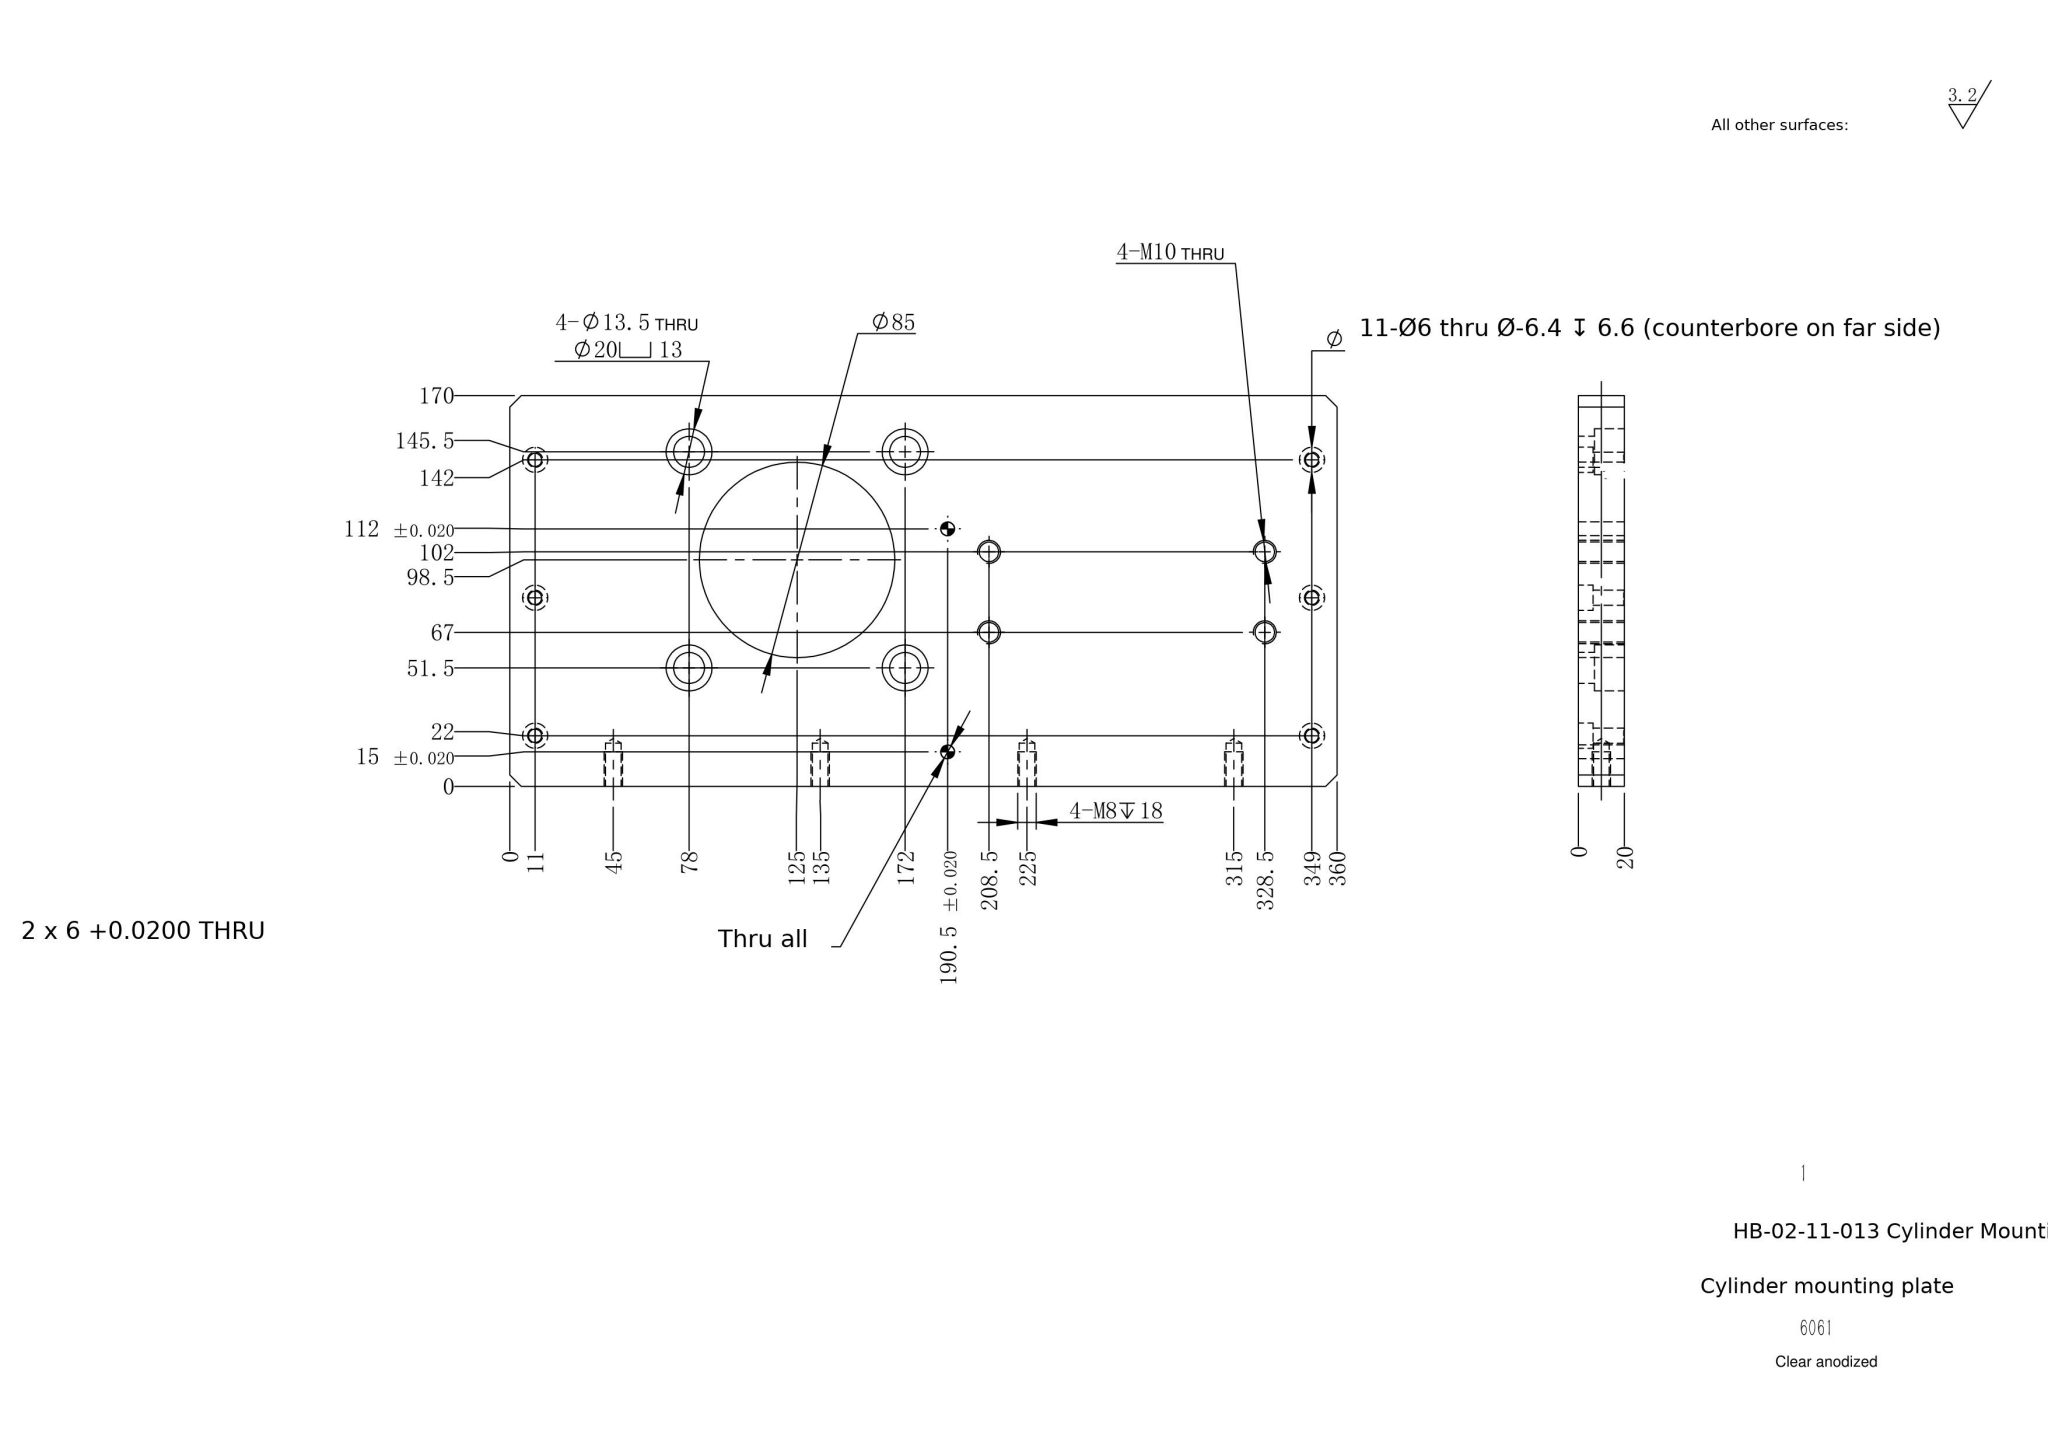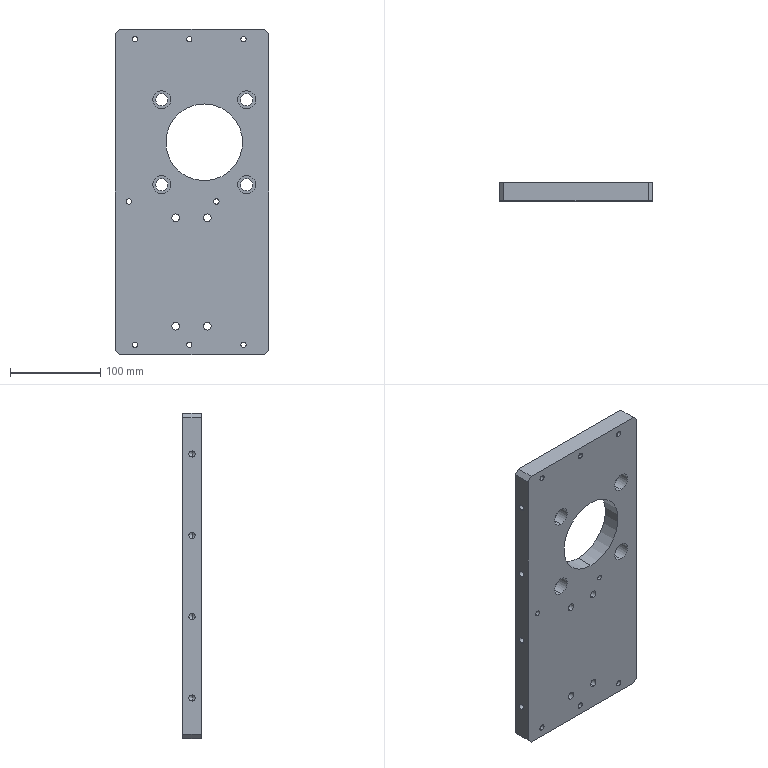Part | SolidWorks | mm | material 6061 | 1 solid | 102 faces | box 170 x 20 x 360 mm | volume 1074238 mm3 | cylinder 62 | cone 20 | plane 20 | commonest cylinder face diameters 11 x12 6.6 x12 8.5 x8 6.8 x8 20 x8 13.5 x8 6 x4 85 x2